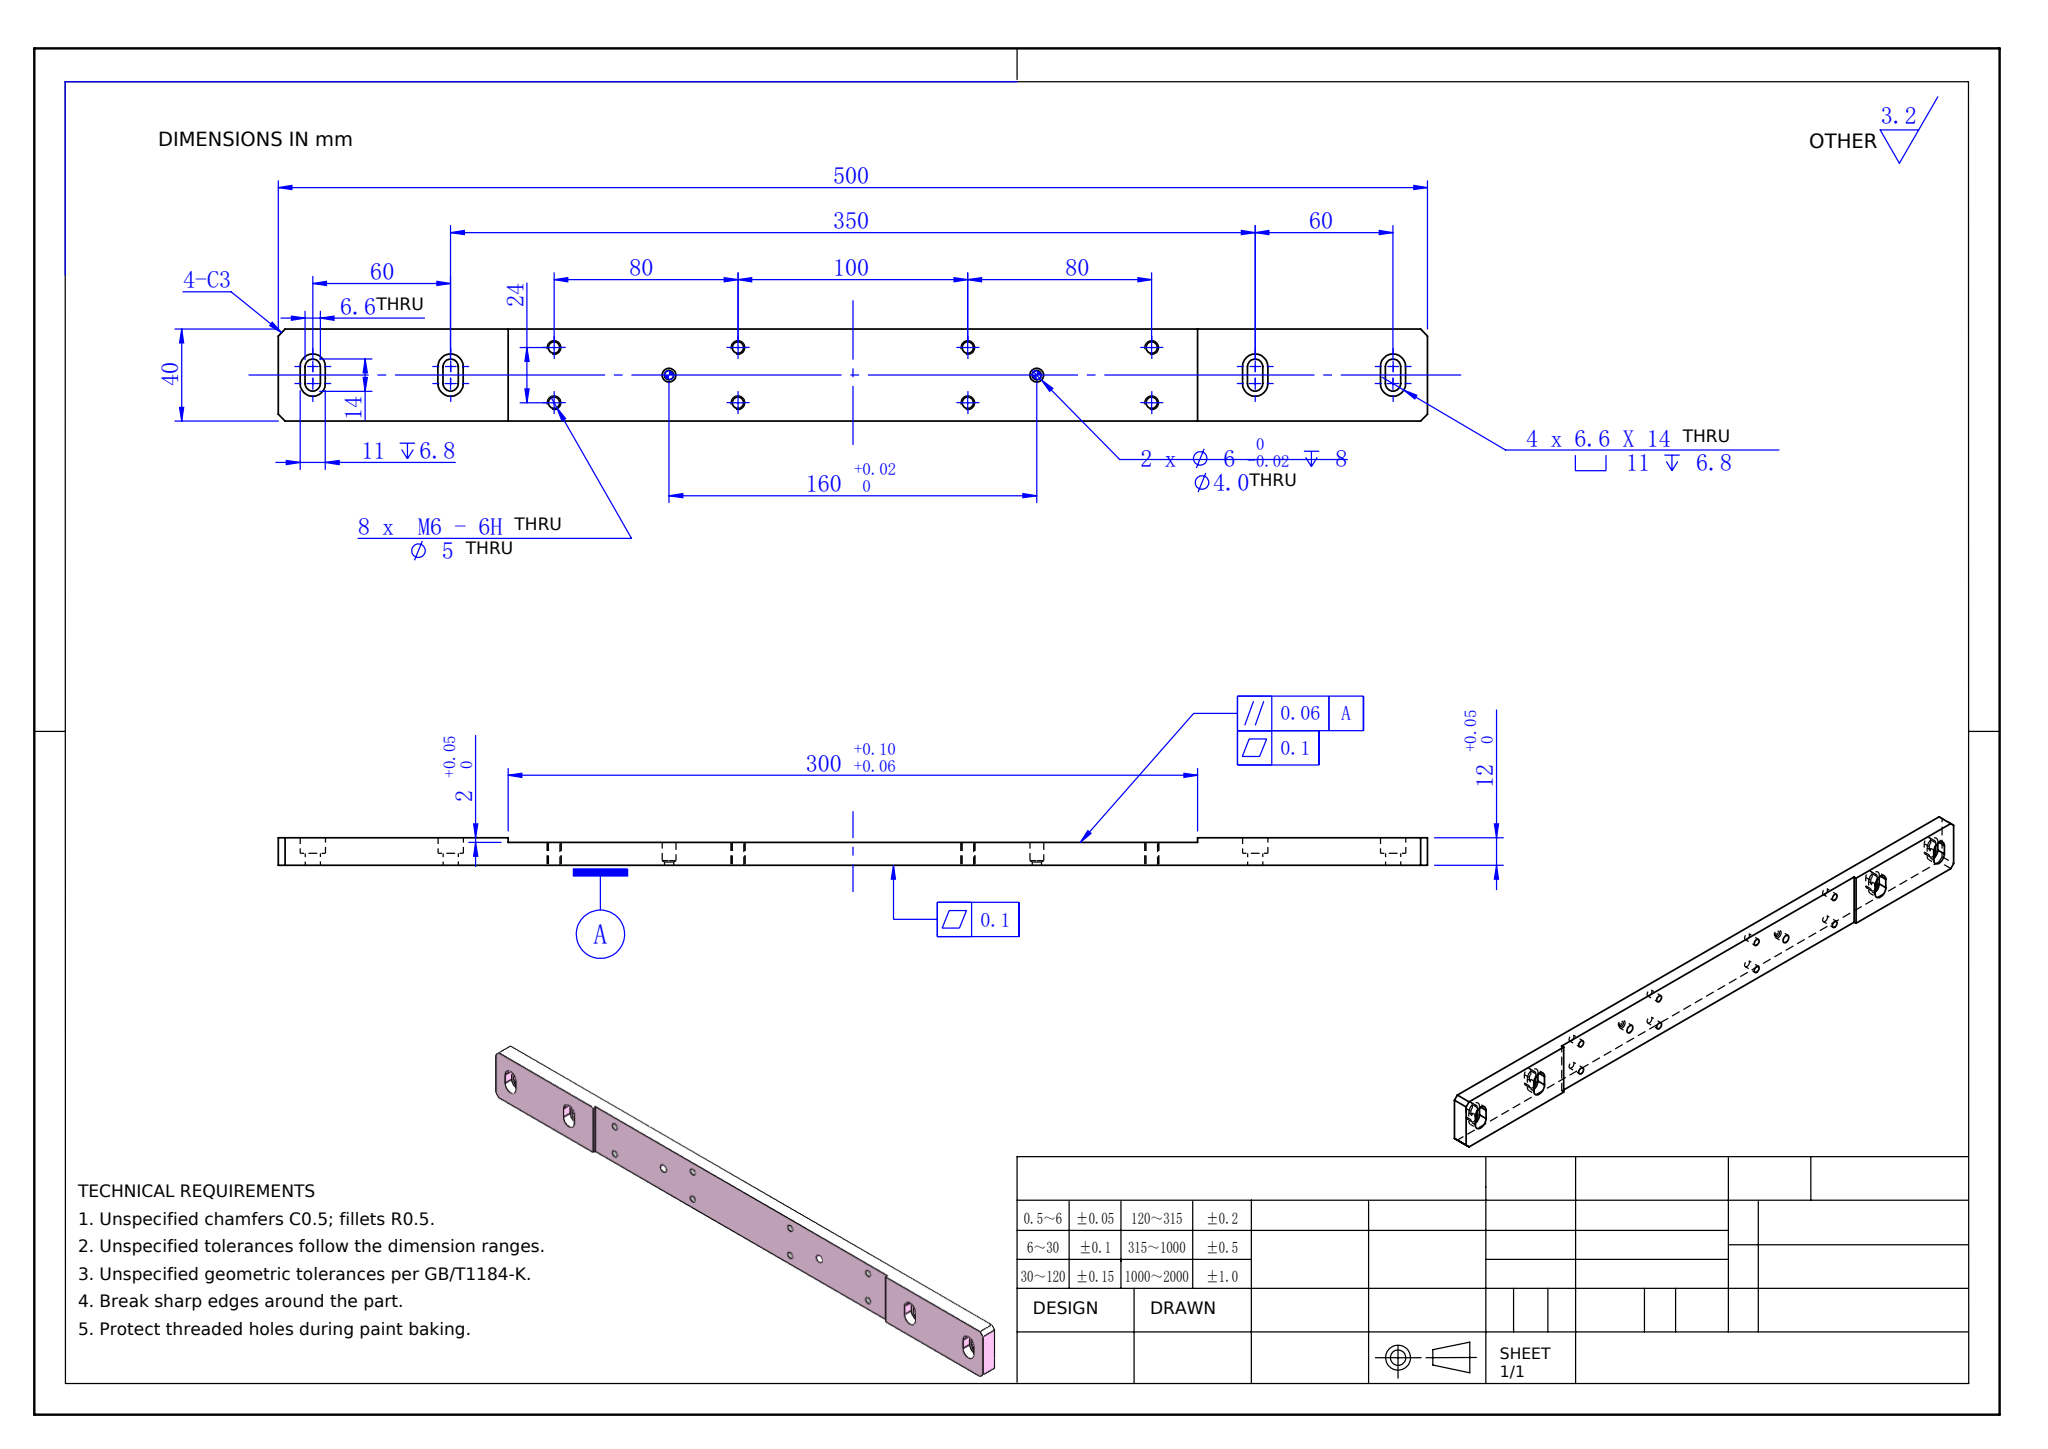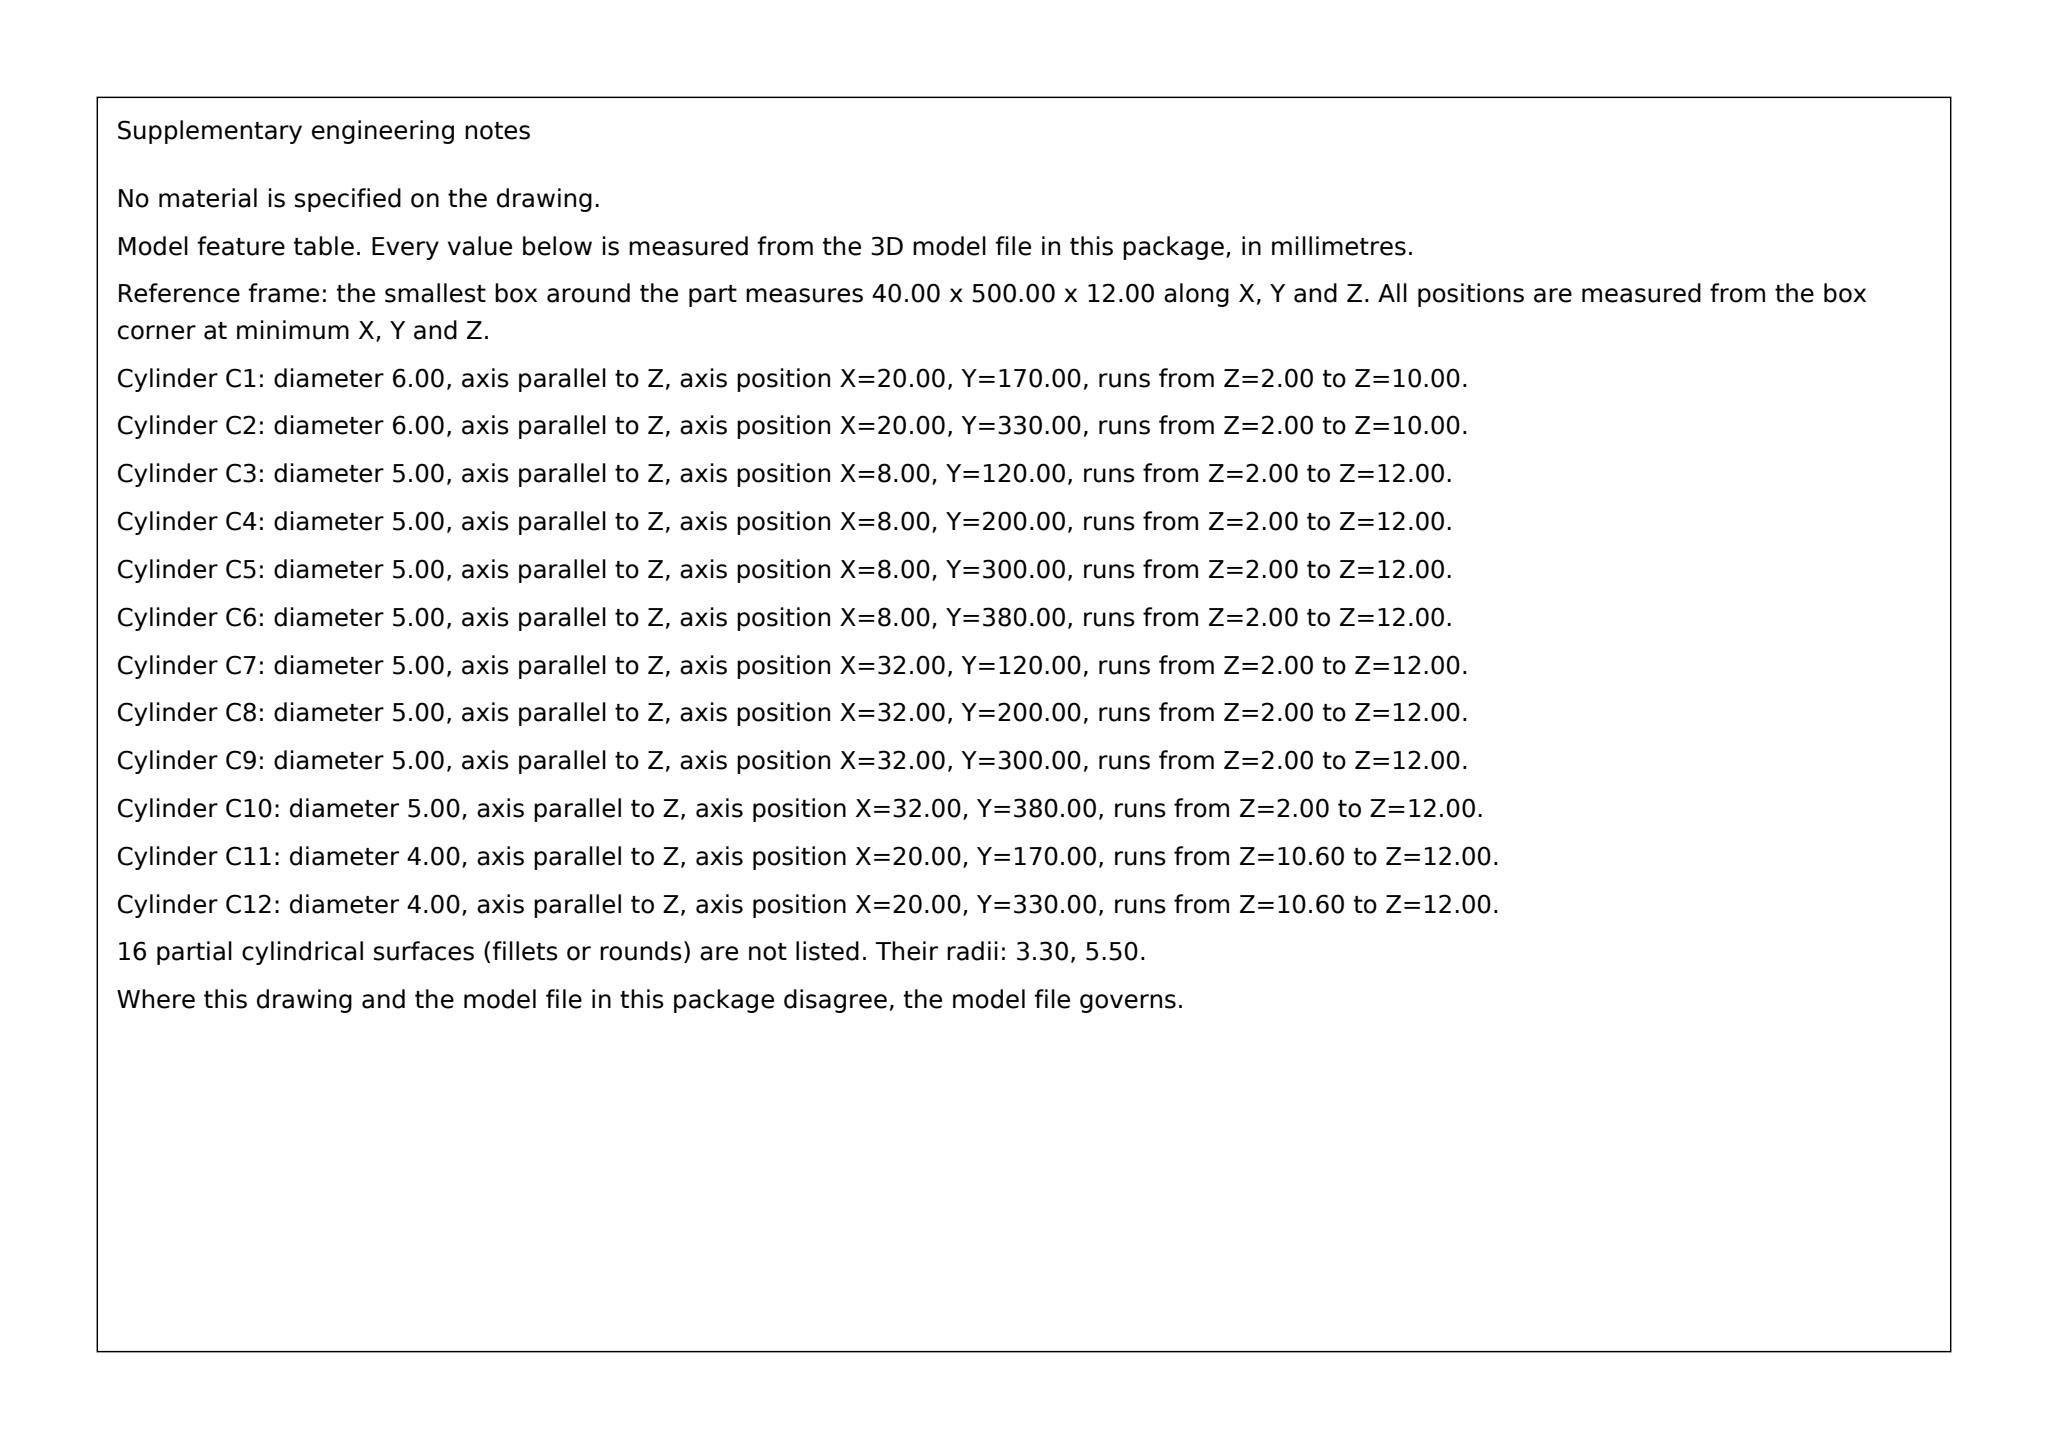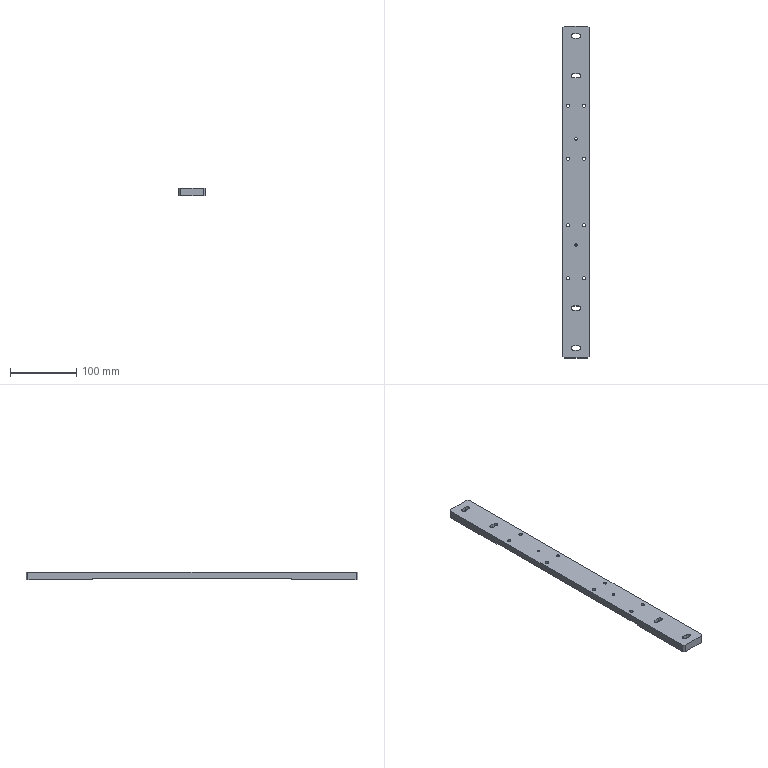Part | SolidWorks | mm | 1 solid | 86 faces | box 40 x 500 x 12 mm | volume 207175 mm3 | cylinder 48 | plane 34 | cone 4 | commonest cylinder face diameters 5 x16 11 x12 6.6 x12 4 x4 6 x4